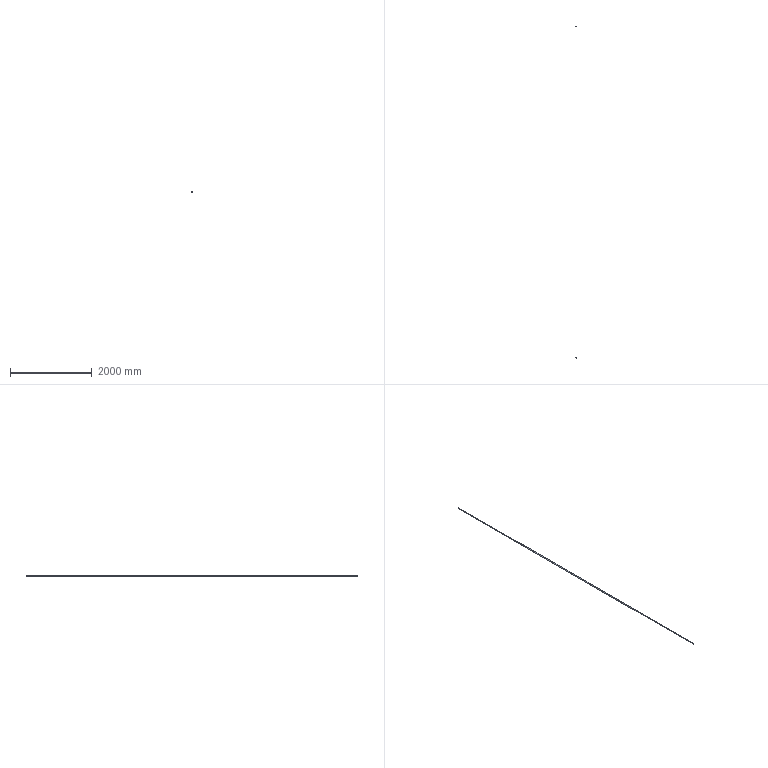Component | NX | 44_3_3 | 1 solid | 4 faces | volume 916088 mm3 | cylinder 2 | plane 2 | commonest cylinder face diameters 20 x1 16 x1